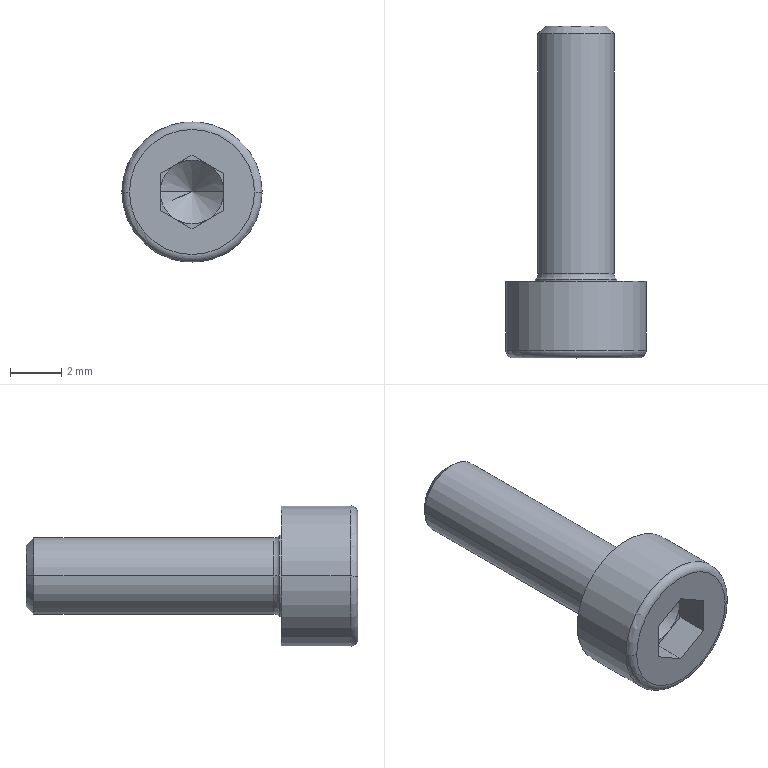Component | SolidWorks | TC_L_12x30_S_0-1_TCL_TCM_12_Screw-1 | 1 solid | 29 faces | box 5.5 x 13 x 5.5 mm | volume 133 mm3 | plane 15 | cylinder 6 | torus 4 | cone 4 | commonest cylinder face diameters 3 x2 3.2 x2 5.5 x2
build123d program:
from build123d import *

# Parameters (mm, degrees)
CUT_EXTRUDE1_DEPTH          = 1.3
SKETCH1_R                   = 2
SKETCH1_R_2                 = 1.6
UNDERHEAD_FILLET_TRIM_DEPTH = 0.4


with BuildPart() as part:
    # Sketch1_2 → Revolve1 (revolve)
    with BuildSketch(Plane.XY, mode=Mode.PRIVATE) as revolve1_sk:
        with BuildLine():
            Line((-3, 0), (-3, 2.45))
            ThreePointArc((-3, 2.45), (-2.912, 2.662), (-2.7, 2.75))
            Line((-2.7, 2.75), (0, 2.75))
            Line((0, 2.75), (0, 1.8))
            ThreePointArc((0, 1.8), (0.08787, 1.588), (0.3, 1.5))
            Line((0.3, 1.5), (9.694, 1.5))
            Line((9.694, 1.5), (10, 1.194))
            Line((10, 1.194), (10, 0))
            Line((10, 0), (-3, 0))
        make_face()
    revolve(revolve1_sk.sketch.rotate(Axis((10, 0, 0), (-1, 0, 0)), 270), axis=Axis((10, 0, 0), (-1, 0, 0)))

    # Sketch2 → Cut-Revolve1 (revolve, cut)
    with BuildSketch(Plane.XY, mode=Mode.PRIVATE) as cut_revolve1_sk:
        Polygon((-3, 0), (-3, 1.25), (-1.7, 1.25), (-0.6, 0), align=None)
    revolve(cut_revolve1_sk.sketch.rotate(Axis((-0.6, 0, 0), (-1, 0, 0)), 270), axis=Axis((-0.6, 0, 0), (-1, 0, 0)), mode=Mode.SUBTRACT)

    # Sketch3 → Cut-Extrude1 (cut)
    with BuildSketch(Plane(origin=(-3, 0, 0), x_dir=(0, 0, -1), z_dir=(1, 0, 0))):
        Polygon((-1.25, 0.7217), (-1.25, -0.7217), (0, -1.443), (1.25, -0.7217), (1.25, 0.7217), (0, 1.443), align=None)
    extrude(amount=CUT_EXTRUDE1_DEPTH, mode=Mode.SUBTRACT)

    # Sketch1 → UnderHead_Fillet_Trim (cut)
    with BuildSketch(Plane(origin=(0, 0, 0), x_dir=(0, 0, -1), z_dir=(1, 0, 0))):
        Circle(SKETCH1_R)
        Circle(SKETCH1_R_2, mode=Mode.SUBTRACT)
    extrude(amount=UNDERHEAD_FILLET_TRIM_DEPTH, mode=Mode.SUBTRACT)


solid = part.part

# Placed as in the assembly
solid = solid.moved(Location((-42, 164.3, 57), (90, 90, 0)))
STEP:
#1=COLOUR_RGB('',0.7922,0.8196,0.9333);
#2=FILL_AREA_STYLE_COLOUR('',#1);
#3=FILL_AREA_STYLE('',(#2));
#4=SURFACE_STYLE_FILL_AREA(#3);
#5=SURFACE_SIDE_STYLE('',(#4));
#6=SURFACE_STYLE_USAGE(.BOTH.,#5);
#7=PRESENTATION_STYLE_ASSIGNMENT((#6));
#8=CARTESIAN_POINT('',(-1.591,6.472,2.244));
#9=VERTEX_POINT('',#8);
#10=CARTESIAN_POINT('',(-1.717,6.472,2.244));
#11=VERTEX_POINT('',#10);
#12=CARTESIAN_POINT('',(-1.654,6.472,2.244));
#13=DIRECTION('',(-0.,1.,0.));
#14=DIRECTION('',(-1.,-0.,0.));
#15=AXIS2_PLACEMENT_3D('',#12,#13,#14);
#16=CIRCLE('',#15,0.06299);
#17=EDGE_CURVE('',#9,#11,#16,.T.);
#18=ORIENTED_EDGE('',*,*,#17,.T.);
#19=CARTESIAN_POINT('',(-1.713,6.48,2.244));
#20=VERTEX_POINT('',#19);
#21=CARTESIAN_POINT('',(-1.724,6.48,2.244));
#22=DIRECTION('',(0.,-0.,1.));
#23=DIRECTION('',(0.,-1.,-0.));
#24=AXIS2_PLACEMENT_3D('',#21,#22,#23);
#25=CIRCLE('',#24,0.01181);
#26=EDGE_CURVE('',#11,#20,#25,.T.);
#27=ORIENTED_EDGE('',*,*,#26,.T.);
#28=CARTESIAN_POINT('',(-1.594,6.48,2.244));
#29=VERTEX_POINT('',#28);
#30=CARTESIAN_POINT('',(-1.654,6.48,2.244));
#31=DIRECTION('',(0.,-1.,-0.));
#32=DIRECTION('',(1.,0.,0.));
#33=AXIS2_PLACEMENT_3D('',#30,#31,#32);
#34=CIRCLE('',#33,0.05906);
#35=EDGE_CURVE('',#20,#29,#34,.T.);
#36=ORIENTED_EDGE('',*,*,#35,.T.);
#37=CARTESIAN_POINT('',(-1.583,6.48,2.244));
#38=DIRECTION('',(-0.,0.,-1.));
#39=DIRECTION('',(0.,1.,0.));
#40=AXIS2_PLACEMENT_3D('',#37,#38,#39);
#41=CIRCLE('',#40,0.01181);
#42=EDGE_CURVE('',#9,#29,#41,.T.);
#43=ORIENTED_EDGE('',*,*,#42,.F.);
#44=EDGE_LOOP('',(#18,#27,#36,#43));
#45=FACE_OUTER_BOUND('',#44,.T.);
#46=CARTESIAN_POINT('',(-1.654,6.48,2.244));
#47=DIRECTION('',(0.,-1.,-0.));
#48=DIRECTION('',(1.,0.,0.));
#49=AXIS2_PLACEMENT_3D('',#46,#47,#48);
#50=TOROIDAL_SURFACE('',#49,0.07087,0.01181);
#51=ADVANCED_FACE('',(#45),#50,.F.);
#52=CARTESIAN_POINT('',(-1.594,6.85,2.244));
#53=VERTEX_POINT('',#52);
#54=CARTESIAN_POINT('',(-1.713,6.85,2.244));
#55=VERTEX_POINT('',#54);
#56=CARTESIAN_POINT('',(-1.654,6.85,2.244));
#57=DIRECTION('',(0.,-1.,-0.));
#58=DIRECTION('',(1.,0.,0.));
#59=AXIS2_PLACEMENT_3D('',#56,#57,#58);
#60=CIRCLE('',#59,0.05906);
#61=EDGE_CURVE('',#53,#55,#60,.T.);
#62=ORIENTED_EDGE('',*,*,#61,.T.);
#63=CARTESIAN_POINT('',(-1.713,6.862,2.244));
#64=DIRECTION('',(0.,-1.,-0.));
#65=VECTOR('',#64,39.37);
#66=LINE('',#63,#65);
#67=EDGE_CURVE('',#55,#20,#66,.T.);
#68=ORIENTED_EDGE('',*,*,#67,.T.);
#69=CARTESIAN_POINT('',(-1.654,6.48,2.244));
#70=DIRECTION('',(0.,-1.,-0.));
#71=DIRECTION('',(1.,0.,0.));
#72=AXIS2_PLACEMENT_3D('',#69,#70,#71);
#73=CIRCLE('',#72,0.05906);
#74=EDGE_CURVE('',#29,#20,#73,.T.);
#75=ORIENTED_EDGE('',*,*,#74,.F.);
#76=CARTESIAN_POINT('',(-1.594,6.862,2.244));
#77=DIRECTION('',(0.,-1.,-0.));
#78=VECTOR('',#77,39.37);
#79=LINE('',#76,#78);
#80=EDGE_CURVE('',#53,#29,#79,.T.);
#81=ORIENTED_EDGE('',*,*,#80,.F.);
#82=EDGE_LOOP('',(#62,#68,#75,#81));
#83=FACE_OUTER_BOUND('',#82,.T.);
#84=CARTESIAN_POINT('',(-1.654,6.862,2.244));
#85=DIRECTION('',(0.,-1.,-0.));
#86=DIRECTION('',(1.,0.,0.));
#87=AXIS2_PLACEMENT_3D('',#84,#85,#86);
#88=CYLINDRICAL_SURFACE('',#87,0.05906);
#89=ADVANCED_FACE('',(#83),#88,.T.);
#90=CARTESIAN_POINT('',(-1.607,6.862,2.244));
#91=VERTEX_POINT('',#90);
#92=CARTESIAN_POINT('',(-1.701,6.862,2.244));
#93=VERTEX_POINT('',#92);
#94=CARTESIAN_POINT('',(-1.654,6.862,2.244));
#95=DIRECTION('',(0.,-1.,-0.));
#96=DIRECTION('',(1.,0.,0.));
#97=AXIS2_PLACEMENT_3D('',#94,#95,#96);
#98=CIRCLE('',#97,0.04699);
#99=EDGE_CURVE('',#91,#93,#98,.T.);
#100=ORIENTED_EDGE('',*,*,#99,.T.);
#101=CARTESIAN_POINT('',(-1.701,6.862,2.244));
#102=DIRECTION('',(-0.7071,-0.7071,-0.));
#103=VECTOR('',#102,39.37);
#104=LINE('',#101,#103);
#105=EDGE_CURVE('',#93,#55,#104,.T.);
#106=ORIENTED_EDGE('',*,*,#105,.T.);
#107=ORIENTED_EDGE('',*,*,#61,.F.);
#108=CARTESIAN_POINT('',(-1.607,6.862,2.244));
#109=DIRECTION('',(0.7071,-0.7071,-0.));
#110=VECTOR('',#109,39.37);
#111=LINE('',#108,#110);
#112=EDGE_CURVE('',#91,#53,#111,.T.);
#113=ORIENTED_EDGE('',*,*,#112,.F.);
#114=EDGE_LOOP('',(#100,#106,#107,#113));
#115=FACE_OUTER_BOUND('',#114,.T.);
#116=CARTESIAN_POINT('',(-1.654,6.862,2.244));
#117=DIRECTION('',(0.,-1.,-0.));
#118=DIRECTION('',(1.,0.,0.));
#119=AXIS2_PLACEMENT_3D('',#116,#117,#118);
#120=CONICAL_SURFACE('',#119,0.04699,0.7854);
#121=ADVANCED_FACE('',(#115),#120,.T.);
#122=CARTESIAN_POINT('',(-1.654,6.472,2.244));
#123=DIRECTION('',(-0.,1.,0.));
#124=DIRECTION('',(-1.,-0.,0.));
#125=AXIS2_PLACEMENT_3D('',#122,#123,#124);
#126=CIRCLE('',#125,0.06299);
#127=EDGE_CURVE('',#11,#9,#126,.T.);
#128=ORIENTED_EDGE('',*,*,#127,.F.);
#129=CARTESIAN_POINT('',(-1.717,6.469,2.244));
#130=VERTEX_POINT('',#129);
#131=CARTESIAN_POINT('',(-1.717,6.484,2.244));
#132=DIRECTION('',(0.,-1.,-0.));
#133=VECTOR('',#132,39.37);
#134=LINE('',#131,#133);
#135=EDGE_CURVE('',#11,#130,#134,.T.);
#136=ORIENTED_EDGE('',*,*,#135,.T.);
#137=CARTESIAN_POINT('',(-1.591,6.469,2.244));
#138=VERTEX_POINT('',#137);
#139=CARTESIAN_POINT('',(-1.654,6.469,2.244));
#140=DIRECTION('',(-0.,1.,0.));
#141=DIRECTION('',(-1.,-0.,0.));
#142=AXIS2_PLACEMENT_3D('',#139,#140,#141);
#143=CIRCLE('',#142,0.06299);
#144=EDGE_CURVE('',#130,#138,#143,.T.);
#145=ORIENTED_EDGE('',*,*,#144,.T.);
#146=CARTESIAN_POINT('',(-1.591,6.484,2.244));
#147=DIRECTION('',(0.,-1.,-0.));
#148=VECTOR('',#147,39.37);
#149=LINE('',#146,#148);
#150=EDGE_CURVE('',#9,#138,#149,.T.);
#151=ORIENTED_EDGE('',*,*,#150,.F.);
#152=EDGE_LOOP('',(#128,#136,#145,#151));
#153=FACE_OUTER_BOUND('',#152,.T.);
#154=CARTESIAN_POINT('',(-1.654,6.484,2.244));
#155=DIRECTION('',(0.,-1.,-0.));
#156=DIRECTION('',(1.,0.,0.));
#157=AXIS2_PLACEMENT_3D('',#154,#155,#156);
#158=CYLINDRICAL_SURFACE('',#157,0.06299);
#159=ADVANCED_FACE('',(#153),#158,.T.);
#160=CARTESIAN_POINT('',(-1.654,6.445,2.244));
#161=VERTEX_POINT('',#160);
#162=CARTESIAN_POINT('',(-1.604,6.402,2.244));
#163=VERTEX_POINT('',#162);
#164=CARTESIAN_POINT('',(-1.654,6.445,2.244));
#165=DIRECTION('',(0.7507,-0.6606,-0.));
#166=VECTOR('',#165,39.37);
#167=LINE('',#164,#166);
#168=EDGE_CURVE('',#161,#163,#167,.T.);
#169=ORIENTED_EDGE('',*,*,#168,.F.);
#170=CARTESIAN_POINT('',(-1.703,6.402,2.244));
#171=VERTEX_POINT('',#170);
#172=CARTESIAN_POINT('',(-1.654,6.445,2.244));
#173=DIRECTION('',(-0.7507,-0.6606,-0.));
#174=VECTOR('',#173,39.37);
#175=LINE('',#172,#174);
#176=EDGE_CURVE('',#161,#171,#175,.T.);
#177=ORIENTED_EDGE('',*,*,#176,.T.);
#178=CARTESIAN_POINT('',(-1.678,6.402,2.201));
#179=VERTEX_POINT('',#178);
#180=CARTESIAN_POINT('',(-1.654,6.402,2.244));
#181=DIRECTION('',(0.,-1.,-0.));
#182=DIRECTION('',(1.,0.,0.));
#183=AXIS2_PLACEMENT_3D('',#180,#181,#182);
#184=CIRCLE('',#183,0.04921);
#185=EDGE_CURVE('',#171,#179,#184,.T.);
#186=ORIENTED_EDGE('',*,*,#185,.T.);
#187=CARTESIAN_POINT('',(-1.629,6.402,2.201));
#188=VERTEX_POINT('',#187);
#189=CARTESIAN_POINT('',(-1.654,6.402,2.244));
#190=DIRECTION('',(0.,-1.,-0.));
#191=DIRECTION('',(1.,0.,0.));
#192=AXIS2_PLACEMENT_3D('',#189,#190,#191);
#193=CIRCLE('',#192,0.04921);
#194=EDGE_CURVE('',#179,#188,#193,.T.);
#195=ORIENTED_EDGE('',*,*,#194,.T.);
#196=CARTESIAN_POINT('',(-1.654,6.402,2.244));
#197=DIRECTION('',(0.,-1.,-0.));
#198=DIRECTION('',(1.,0.,0.));
#199=AXIS2_PLACEMENT_3D('',#196,#197,#198);
#200=CIRCLE('',#199,0.04921);
#201=EDGE_CURVE('',#188,#163,#200,.T.);
#202=ORIENTED_EDGE('',*,*,#201,.T.);
#203=EDGE_LOOP('',(#169,#177,#186,#195,#202));
#204=FACE_OUTER_BOUND('',#203,.T.);
#205=CARTESIAN_POINT('',(-1.654,-32.925,2.244));
#206=DIRECTION('',(0.,-1.,-0.));
#207=DIRECTION('',(1.,0.,-0.));
#208=AXIS2_PLACEMENT_3D('',#205,#206,#207);
#209=CONICAL_SURFACE('',#208,44.739,0.8491);
#210=ADVANCED_FACE('',(#204),#209,.F.);
#211=CARTESIAN_POINT('',(-1.545,6.469,2.244));
#212=VERTEX_POINT('',#211);
#213=CARTESIAN_POINT('',(-1.762,6.469,2.244));
#214=VERTEX_POINT('',#213);
#215=CARTESIAN_POINT('',(-1.654,6.469,2.244));
#216=DIRECTION('',(0.,-1.,-0.));
#217=DIRECTION('',(1.,0.,0.));
#218=AXIS2_PLACEMENT_3D('',#215,#216,#217);
#219=CIRCLE('',#218,0.1083);
#220=EDGE_CURVE('',#212,#214,#219,.T.);
#221=ORIENTED_EDGE('',*,*,#220,.T.);
#222=CARTESIAN_POINT('',(-1.762,6.362,2.244));
#223=VERTEX_POINT('',#222);
#224=CARTESIAN_POINT('',(-1.762,6.862,2.244));
#225=DIRECTION('',(0.,-1.,-0.));
#226=VECTOR('',#225,39.37);
#227=LINE('',#224,#226);
#228=EDGE_CURVE('',#214,#223,#227,.T.);
#229=ORIENTED_EDGE('',*,*,#228,.T.);
#230=CARTESIAN_POINT('',(-1.545,6.362,2.244));
#231=VERTEX_POINT('',#230);
#232=CARTESIAN_POINT('',(-1.654,6.362,2.244));
#233=DIRECTION('',(0.,-1.,-0.));
#234=DIRECTION('',(1.,0.,0.));
#235=AXIS2_PLACEMENT_3D('',#232,#233,#234);
#236=CIRCLE('',#235,0.1083);
#237=EDGE_CURVE('',#231,#223,#236,.T.);
#238=ORIENTED_EDGE('',*,*,#237,.F.);
#239=CARTESIAN_POINT('',(-1.545,6.862,2.244));
#240=DIRECTION('',(0.,-1.,-0.));
#241=VECTOR('',#240,39.37);
#242=LINE('',#239,#241);
#243=EDGE_CURVE('',#212,#231,#242,.T.);
#244=ORIENTED_EDGE('',*,*,#243,.F.);
#245=EDGE_LOOP('',(#221,#229,#238,#244));
#246=FACE_OUTER_BOUND('',#245,.T.);
#247=CARTESIAN_POINT('',(-1.654,6.862,2.244));
#248=DIRECTION('',(0.,-1.,-0.));
#249=DIRECTION('',(1.,0.,0.));
#250=AXIS2_PLACEMENT_3D('',#247,#248,#249);
#251=CYLINDRICAL_SURFACE('',#250,0.1083);
#252=ADVANCED_FACE('',(#246),#251,.T.);
#253=ORIENTED_EDGE('',*,*,#237,.T.);
#254=CARTESIAN_POINT('',(-1.75,6.35,2.244));
#255=VERTEX_POINT('',#254);
#256=CARTESIAN_POINT('',(-1.75,6.362,2.244));
#257=DIRECTION('',(0.,-0.,1.));
#258=DIRECTION('',(0.,-1.,-0.));
#259=AXIS2_PLACEMENT_3D('',#256,#257,#258);
#260=CIRCLE('',#259,0.01181);
#261=EDGE_CURVE('',#223,#255,#260,.T.);
#262=ORIENTED_EDGE('',*,*,#261,.T.);
#263=CARTESIAN_POINT('',(-1.557,6.35,2.244));
#264=VERTEX_POINT('',#263);
#265=CARTESIAN_POINT('',(-1.654,6.35,2.244));
#266=DIRECTION('',(0.,-1.,-0.));
#267=DIRECTION('',(1.,0.,0.));
#268=AXIS2_PLACEMENT_3D('',#265,#266,#267);
#269=CIRCLE('',#268,0.09646);
#270=EDGE_CURVE('',#264,#255,#269,.T.);
#271=ORIENTED_EDGE('',*,*,#270,.F.);
#272=CARTESIAN_POINT('',(-1.557,6.362,2.244));
#273=DIRECTION('',(-0.,0.,-1.));
#274=DIRECTION('',(0.,1.,0.));
#275=AXIS2_PLACEMENT_3D('',#272,#273,#274);
#276=CIRCLE('',#275,0.01181);
#277=EDGE_CURVE('',#231,#264,#276,.T.);
#278=ORIENTED_EDGE('',*,*,#277,.F.);
#279=EDGE_LOOP('',(#253,#262,#271,#278));
#280=FACE_OUTER_BOUND('',#279,.T.);
#281=CARTESIAN_POINT('',(-1.654,6.362,2.244));
#282=DIRECTION('',(0.,-1.,-0.));
#283=DIRECTION('',(1.,0.,0.));
#284=AXIS2_PLACEMENT_3D('',#281,#282,#283);
#285=TOROIDAL_SURFACE('',#284,0.09646,0.01181);
#286=ADVANCED_FACE('',(#280),#285,.T.);
#287=ORIENTED_EDGE('',*,*,#270,.T.);
#288=CARTESIAN_POINT('',(-1.654,6.35,2.244));
#289=DIRECTION('',(0.,-1.,-0.));
#290=DIRECTION('',(1.,0.,0.));
#291=AXIS2_PLACEMENT_3D('',#288,#289,#290);
#292=CIRCLE('',#291,0.09646);
#293=EDGE_CURVE('',#255,#264,#292,.T.);
#294=ORIENTED_EDGE('',*,*,#293,.T.);
#295=EDGE_LOOP('',(#287,#294));
#296=FACE_OUTER_BOUND('',#295,.T.);
#297=CARTESIAN_POINT('',(-1.604,6.35,2.216));
#298=VERTEX_POINT('',#297);
#299=CARTESIAN_POINT('',(-1.654,6.35,2.187));
#300=VERTEX_POINT('',#299);
#301=CARTESIAN_POINT('',(-1.604,6.35,2.216));
#302=DIRECTION('',(-0.866,-0.,-0.5));
#303=VECTOR('',#302,39.37);
#304=LINE('',#301,#303);
#305=EDGE_CURVE('',#298,#300,#304,.T.);
#306=ORIENTED_EDGE('',*,*,#305,.T.);
#307=CARTESIAN_POINT('',(-1.703,6.35,2.216));
#308=VERTEX_POINT('',#307);
#309=CARTESIAN_POINT('',(-1.654,6.35,2.187));
#310=DIRECTION('',(-0.866,-0.,0.5));
#311=VECTOR('',#310,39.37);
#312=LINE('',#309,#311);
#313=EDGE_CURVE('',#300,#308,#312,.T.);
#314=ORIENTED_EDGE('',*,*,#313,.T.);
#315=CARTESIAN_POINT('',(-1.703,6.35,2.273));
#316=VERTEX_POINT('',#315);
#317=CARTESIAN_POINT('',(-1.703,6.35,2.216));
#318=DIRECTION('',(0.,-0.,1.));
#319=VECTOR('',#318,39.37);
#320=LINE('',#317,#319);
#321=EDGE_CURVE('',#308,#316,#320,.T.);
#322=ORIENTED_EDGE('',*,*,#321,.T.);
#323=CARTESIAN_POINT('',(-1.654,6.35,2.301));
#324=VERTEX_POINT('',#323);
#325=CARTESIAN_POINT('',(-1.703,6.35,2.273));
#326=DIRECTION('',(0.866,0.,0.5));
#327=VECTOR('',#326,39.37);
#328=LINE('',#325,#327);
#329=EDGE_CURVE('',#316,#324,#328,.T.);
#330=ORIENTED_EDGE('',*,*,#329,.T.);
#331=CARTESIAN_POINT('',(-1.604,6.35,2.273));
#332=VERTEX_POINT('',#331);
#333=CARTESIAN_POINT('',(-1.654,6.35,2.301));
#334=DIRECTION('',(0.866,0.,-0.5));
#335=VECTOR('',#334,39.37);
#336=LINE('',#333,#335);
#337=EDGE_CURVE('',#324,#332,#336,.T.);
#338=ORIENTED_EDGE('',*,*,#337,.T.);
#339=CARTESIAN_POINT('',(-1.604,6.35,2.273));
#340=DIRECTION('',(-0.,0.,-1.));
#341=VECTOR('',#340,39.37);
#342=LINE('',#339,#341);
#343=EDGE_CURVE('',#332,#298,#342,.T.);
#344=ORIENTED_EDGE('',*,*,#343,.T.);
#345=EDGE_LOOP('',(#306,#314,#322,#330,#338,#344));
#346=FACE_BOUND('',#345,.T.);
#347=CARTESIAN_POINT('',(-1.654,6.35,2.244));
#348=DIRECTION('',(-0.,1.,0.));
#349=DIRECTION('',(-1.,-0.,0.));
#350=AXIS2_PLACEMENT_3D('',#347,#348,#349);
#351=PLANE('',#350);
#352=ADVANCED_FACE('',(#296,#346),#351,.F.);
#353=ORIENTED_EDGE('',*,*,#261,.F.);
#354=CARTESIAN_POINT('',(-1.654,6.362,2.244));
#355=DIRECTION('',(0.,-1.,-0.));
#356=DIRECTION('',(1.,0.,0.));
#357=AXIS2_PLACEMENT_3D('',#354,#355,#356);
#358=CIRCLE('',#357,0.1083);
#359=EDGE_CURVE('',#223,#231,#358,.T.);
#360=ORIENTED_EDGE('',*,*,#359,.T.);
#361=ORIENTED_EDGE('',*,*,#277,.T.);
#362=ORIENTED_EDGE('',*,*,#293,.F.);
#363=EDGE_LOOP('',(#353,#360,#361,#362));
#364=FACE_OUTER_BOUND('',#363,.T.);
#365=CARTESIAN_POINT('',(-1.654,6.362,2.244));
#366=DIRECTION('',(0.,-1.,-0.));
#367=DIRECTION('',(1.,0.,0.));
#368=AXIS2_PLACEMENT_3D('',#365,#366,#367);
#369=TOROIDAL_SURFACE('',#368,0.09646,0.01181);
#370=ADVANCED_FACE('',(#364),#369,.T.);
#371=ORIENTED_EDGE('',*,*,#228,.F.);
#372=CARTESIAN_POINT('',(-1.654,6.469,2.244));
#373=DIRECTION('',(0.,-1.,-0.));
#374=DIRECTION('',(1.,0.,0.));
#375=AXIS2_PLACEMENT_3D('',#372,#373,#374);
#376=CIRCLE('',#375,0.1083);
#377=EDGE_CURVE('',#214,#212,#376,.T.);
#378=ORIENTED_EDGE('',*,*,#377,.T.);
#379=ORIENTED_EDGE('',*,*,#243,.T.);
#380=ORIENTED_EDGE('',*,*,#359,.F.);
#381=EDGE_LOOP('',(#371,#378,#379,#380));
#382=FACE_OUTER_BOUND('',#381,.T.);
#383=CARTESIAN_POINT('',(-1.654,6.862,2.244));
#384=DIRECTION('',(0.,-1.,-0.));
#385=DIRECTION('',(1.,0.,0.));
#386=AXIS2_PLACEMENT_3D('',#383,#384,#385);
#387=CYLINDRICAL_SURFACE('',#386,0.1083);
#388=ADVANCED_FACE('',(#382),#387,.T.);
#389=ORIENTED_EDGE('',*,*,#220,.F.);
#390=ORIENTED_EDGE('',*,*,#377,.F.);
#391=EDGE_LOOP('',(#389,#390));
#392=FACE_OUTER_BOUND('',#391,.T.);
#393=CARTESIAN_POINT('',(-1.654,6.469,2.244));
#394=DIRECTION('',(-0.,1.,0.));
#395=DIRECTION('',(-1.,-0.,0.));
#396=AXIS2_PLACEMENT_3D('',#393,#394,#395);
#397=CIRCLE('',#396,0.06299);
#398=EDGE_CURVE('',#138,#130,#397,.T.);
#399=ORIENTED_EDGE('',*,*,#398,.F.);
#400=ORIENTED_EDGE('',*,*,#144,.F.);
#401=EDGE_LOOP('',(#399,#400));
#402=FACE_BOUND('',#401,.T.);
#403=CARTESIAN_POINT('',(-1.654,6.469,2.352));
#404=DIRECTION('',(0.,-1.,-0.));
#405=DIRECTION('',(1.,0.,-0.));
#406=AXIS2_PLACEMENT_3D('',#403,#404,#405);
#407=PLANE('',#406);
#408=ADVANCED_FACE('',(#392,#402),#407,.F.);
#409=CARTESIAN_POINT('',(-1.654,6.402,2.301));
#410=VERTEX_POINT('',#409);
#411=CARTESIAN_POINT('',(-1.629,6.402,2.287));
#412=VERTEX_POINT('',#411);
#413=CARTESIAN_POINT('',(-1.654,6.402,2.301));
#414=DIRECTION('',(0.866,0.,-0.5));
#415=VECTOR('',#414,39.37);
#416=LINE('',#413,#415);
#417=EDGE_CURVE('',#410,#412,#416,.T.);
#418=ORIENTED_EDGE('',*,*,#417,.T.);
#419=CARTESIAN_POINT('',(-1.604,6.402,2.273));
#420=VERTEX_POINT('',#419);
#421=CARTESIAN_POINT('',(-1.654,6.402,2.301));
#422=DIRECTION('',(0.866,0.,-0.5));
#423=VECTOR('',#422,39.37);
#424=LINE('',#421,#423);
#425=EDGE_CURVE('',#412,#420,#424,.T.);
#426=ORIENTED_EDGE('',*,*,#425,.T.);
#427=CARTESIAN_POINT('',(-1.604,6.402,2.273));
#428=DIRECTION('',(0.,-1.,-0.));
#429=VECTOR('',#428,39.37);
#430=LINE('',#427,#429);
#431=EDGE_CURVE('',#420,#332,#430,.T.);
#432=ORIENTED_EDGE('',*,*,#431,.T.);
#433=ORIENTED_EDGE('',*,*,#337,.F.);
#434=CARTESIAN_POINT('',(-1.654,6.402,2.301));
#435=DIRECTION('',(0.,-1.,-0.));
#436=VECTOR('',#435,39.37);
#437=LINE('',#434,#436);
#438=EDGE_CURVE('',#410,#324,#437,.T.);
#439=ORIENTED_EDGE('',*,*,#438,.F.);
#440=EDGE_LOOP('',(#418,#426,#432,#433,#439));
#441=FACE_OUTER_BOUND('',#440,.T.);
#442=CARTESIAN_POINT('',(-1.654,6.402,2.301));
#443=DIRECTION('',(-0.5,0.,-0.866));
#444=DIRECTION('',(-0.866,-0.,0.5));
#445=AXIS2_PLACEMENT_3D('',#442,#443,#444);
#446=PLANE('',#445);
#447=ADVANCED_FACE('',(#441),#446,.T.);
#448=CARTESIAN_POINT('',(-1.604,6.402,2.273));
#449=DIRECTION('',(-0.,0.,-1.));
#450=VECTOR('',#449,39.37);
#451=LINE('',#448,#450);
#452=EDGE_CURVE('',#420,#163,#451,.T.);
#453=ORIENTED_EDGE('',*,*,#452,.T.);
#454=CARTESIAN_POINT('',(-1.604,6.402,2.216));
#455=VERTEX_POINT('',#454);
#456=CARTESIAN_POINT('',(-1.604,6.402,2.273));
#457=DIRECTION('',(-0.,0.,-1.));
#458=VECTOR('',#457,39.37);
#459=LINE('',#456,#458);
#460=EDGE_CURVE('',#163,#455,#459,.T.);
#461=ORIENTED_EDGE('',*,*,#460,.T.);
#462=CARTESIAN_POINT('',(-1.604,6.402,2.216));
#463=DIRECTION('',(0.,-1.,-0.));
#464=VECTOR('',#463,39.37);
#465=LINE('',#462,#464);
#466=EDGE_CURVE('',#455,#298,#465,.T.);
#467=ORIENTED_EDGE('',*,*,#466,.T.);
#468=ORIENTED_EDGE('',*,*,#343,.F.);
#469=ORIENTED_EDGE('',*,*,#431,.F.);
#470=EDGE_LOOP('',(#453,#461,#467,#468,#469));
#471=FACE_OUTER_BOUND('',#470,.T.);
#472=CARTESIAN_POINT('',(-1.604,6.402,2.273));
#473=DIRECTION('',(-1.,-0.,0.));
#474=DIRECTION('',(0.,-1.,-0.));
#475=AXIS2_PLACEMENT_3D('',#472,#473,#474);
#476=PLANE('',#475);
#477=ADVANCED_FACE('',(#471),#476,.T.);
#478=CARTESIAN_POINT('',(-1.604,6.402,2.216));
#479=DIRECTION('',(-0.866,-0.,-0.5));
#480=VECTOR('',#479,39.37);
#481=LINE('',#478,#480);
#482=EDGE_CURVE('',#455,#188,#481,.T.);
#483=ORIENTED_EDGE('',*,*,#482,.T.);
#484=CARTESIAN_POINT('',(-1.654,6.402,2.187));
#485=VERTEX_POINT('',#484);
#486=CARTESIAN_POINT('',(-1.604,6.402,2.216));
#487=DIRECTION('',(-0.866,-0.,-0.5));
#488=VECTOR('',#487,39.37);
#489=LINE('',#486,#488);
#490=EDGE_CURVE('',#188,#485,#489,.T.);
#491=ORIENTED_EDGE('',*,*,#490,.T.);
#492=CARTESIAN_POINT('',(-1.654,6.402,2.187));
#493=DIRECTION('',(0.,-1.,-0.));
#494=VECTOR('',#493,39.37);
#495=LINE('',#492,#494);
#496=EDGE_CURVE('',#485,#300,#495,.T.);
#497=ORIENTED_EDGE('',*,*,#496,.T.);
#498=ORIENTED_EDGE('',*,*,#305,.F.);
#499=ORIENTED_EDGE('',*,*,#466,.F.);
#500=EDGE_LOOP('',(#483,#491,#497,#498,#499));
#501=FACE_OUTER_BOUND('',#500,.T.);
#502=CARTESIAN_POINT('',(-1.604,6.402,2.216));
#503=DIRECTION('',(-0.5,-0.,0.866));
#504=DIRECTION('',(0.866,0.,0.5));
#505=AXIS2_PLACEMENT_3D('',#502,#503,#504);
#506=PLANE('',#505);
#507=ADVANCED_FACE('',(#501),#506,.T.);
#508=CARTESIAN_POINT('',(-1.654,6.402,2.187));
#509=DIRECTION('',(-0.866,-0.,0.5));
#510=VECTOR('',#509,39.37);
#511=LINE('',#508,#510);
#512=EDGE_CURVE('',#485,#179,#511,.T.);
#513=ORIENTED_EDGE('',*,*,#512,.T.);
#514=CARTESIAN_POINT('',(-1.703,6.402,2.216));
#515=VERTEX_POINT('',#514);
#516=CARTESIAN_POINT('',(-1.654,6.402,2.187));
#517=DIRECTION('',(-0.866,-0.,0.5));
#518=VECTOR('',#517,39.37);
#519=LINE('',#516,#518);
#520=EDGE_CURVE('',#179,#515,#519,.T.);
#521=ORIENTED_EDGE('',*,*,#520,.T.);
#522=CARTESIAN_POINT('',(-1.703,6.402,2.216));
#523=DIRECTION('',(0.,-1.,-0.));
#524=VECTOR('',#523,39.37);
#525=LINE('',#522,#524);
#526=EDGE_CURVE('',#515,#308,#525,.T.);
#527=ORIENTED_EDGE('',*,*,#526,.T.);
#528=ORIENTED_EDGE('',*,*,#313,.F.);
#529=ORIENTED_EDGE('',*,*,#496,.F.);
#530=EDGE_LOOP('',(#513,#521,#527,#528,#529));
#531=FACE_OUTER_BOUND('',#530,.T.);
#532=CARTESIAN_POINT('',(-1.654,6.402,2.187));
#533=DIRECTION('',(0.5,-0.,0.866));
#534=DIRECTION('',(0.866,0.,-0.5));
#535=AXIS2_PLACEMENT_3D('',#532,#533,#534);
#536=PLANE('',#535);
#537=ADVANCED_FACE('',(#531),#536,.T.);
#538=CARTESIAN_POINT('',(-1.703,6.402,2.216));
#539=DIRECTION('',(0.,-0.,1.));
#540=VECTOR('',#539,39.37);
#541=LINE('',#538,#540);
#542=EDGE_CURVE('',#515,#171,#541,.T.);
#543=ORIENTED_EDGE('',*,*,#542,.T.);
#544=CARTESIAN_POINT('',(-1.703,6.402,2.273));
#545=VERTEX_POINT('',#544);
#546=CARTESIAN_POINT('',(-1.703,6.402,2.216));
#547=DIRECTION('',(0.,-0.,1.));
#548=VECTOR('',#547,39.37);
#549=LINE('',#546,#548);
#550=EDGE_CURVE('',#171,#545,#549,.T.);
#551=ORIENTED_EDGE('',*,*,#550,.T.);
#552=CARTESIAN_POINT('',(-1.703,6.402,2.273));
#553=DIRECTION('',(0.,-1.,-0.));
#554=VECTOR('',#553,39.37);
#555=LINE('',#552,#554);
#556=EDGE_CURVE('',#545,#316,#555,.T.);
#557=ORIENTED_EDGE('',*,*,#556,.T.);
#558=ORIENTED_EDGE('',*,*,#321,.F.);
#559=ORIENTED_EDGE('',*,*,#526,.F.);
#560=EDGE_LOOP('',(#543,#551,#557,#558,#559));
#561=FACE_OUTER_BOUND('',#560,.T.);
#562=CARTESIAN_POINT('',(-1.703,6.402,2.216));
#563=DIRECTION('',(1.,0.,-0.));
#564=DIRECTION('',(-0.,1.,0.));
#565=AXIS2_PLACEMENT_3D('',#562,#563,#564);
#566=PLANE('',#565);
#567=ADVANCED_FACE('',(#561),#566,.T.);
#568=CARTESIAN_POINT('',(-1.678,6.402,2.287));
#569=VERTEX_POINT('',#568);
#570=CARTESIAN_POINT('',(-1.703,6.402,2.273));
#571=DIRECTION('',(0.866,0.,0.5));
#572=VECTOR('',#571,39.37);
#573=LINE('',#570,#572);
#574=EDGE_CURVE('',#545,#569,#573,.T.);
#575=ORIENTED_EDGE('',*,*,#574,.T.);
#576=CARTESIAN_POINT('',(-1.703,6.402,2.273));
#577=DIRECTION('',(0.866,0.,0.5));
#578=VECTOR('',#577,39.37);
#579=LINE('',#576,#578);
#580=EDGE_CURVE('',#569,#410,#579,.T.);
#581=ORIENTED_EDGE('',*,*,#580,.T.);
#582=ORIENTED_EDGE('',*,*,#438,.T.);
#583=ORIENTED_EDGE('',*,*,#329,.F.);
#584=ORIENTED_EDGE('',*,*,#556,.F.);
#585=EDGE_LOOP('',(#575,#581,#582,#583,#584));
#586=FACE_OUTER_BOUND('',#585,.T.);
#587=CARTESIAN_POINT('',(-1.703,6.402,2.273));
#588=DIRECTION('',(0.5,0.,-0.866));
#589=DIRECTION('',(-0.866,-0.,-0.5));
#590=AXIS2_PLACEMENT_3D('',#587,#588,#589);
#591=PLANE('',#590);
#592=ADVANCED_FACE('',(#586),#591,.T.);
#593=CARTESIAN_POINT('',(-1.654,6.402,2.244));
#594=DIRECTION('',(0.,-1.,-0.));
#595=DIRECTION('',(1.,0.,0.));
#596=AXIS2_PLACEMENT_3D('',#593,#594,#595);
#597=CIRCLE('',#596,0.04921);
#598=EDGE_CURVE('',#569,#171,#597,.T.);
#599=ORIENTED_EDGE('',*,*,#598,.F.);
#600=ORIENTED_EDGE('',*,*,#574,.F.);
#601=ORIENTED_EDGE('',*,*,#550,.F.);
#602=EDGE_LOOP('',(#599,#600,#601));
#603=FACE_OUTER_BOUND('',#602,.T.);
#604=CARTESIAN_POINT('',(-1.654,6.402,2.244));
#605=DIRECTION('',(-0.,1.,0.));
#606=DIRECTION('',(-1.,-0.,0.));
#607=AXIS2_PLACEMENT_3D('',#604,#605,#606);
#608=PLANE('',#607);
#609=ADVANCED_FACE('',(#603),#608,.F.);
#610=CARTESIAN_POINT('',(-1.654,6.402,2.244));
#611=DIRECTION('',(0.,-1.,-0.));
#612=DIRECTION('',(1.,0.,0.));
#613=AXIS2_PLACEMENT_3D('',#610,#611,#612);
#614=CIRCLE('',#613,0.04921);
#615=EDGE_CURVE('',#412,#569,#614,.T.);
#616=ORIENTED_EDGE('',*,*,#615,.F.);
#617=ORIENTED_EDGE('',*,*,#417,.F.);
#618=ORIENTED_EDGE('',*,*,#580,.F.);
#619=EDGE_LOOP('',(#616,#617,#618));
#620=FACE_OUTER_BOUND('',#619,.T.);
#621=CARTESIAN_POINT('',(-1.654,6.402,2.244));
#622=DIRECTION('',(-0.,1.,0.));
#623=DIRECTION('',(-1.,-0.,0.));
#624=AXIS2_PLACEMENT_3D('',#621,#622,#623);
#625=PLANE('',#624);
#626=ADVANCED_FACE('',(#620),#625,.F.);
#627=CARTESIAN_POINT('',(-1.654,6.402,2.244));
#628=DIRECTION('',(0.,-1.,-0.));
#629=DIRECTION('',(1.,0.,0.));
#630=AXIS2_PLACEMENT_3D('',#627,#628,#629);
#631=CIRCLE('',#630,0.04921);
#632=EDGE_CURVE('',#163,#412,#631,.T.);
#633=ORIENTED_EDGE('',*,*,#632,.F.);
#634=ORIENTED_EDGE('',*,*,#452,.F.);
#635=ORIENTED_EDGE('',*,*,#425,.F.);
#636=EDGE_LOOP('',(#633,#634,#635));
#637=FACE_OUTER_BOUND('',#636,.T.);
#638=CARTESIAN_POINT('',(-1.654,6.402,2.244));
#639=DIRECTION('',(-0.,1.,0.));
#640=DIRECTION('',(-1.,-0.,0.));
#641=AXIS2_PLACEMENT_3D('',#638,#639,#640);
#642=PLANE('',#641);
#643=ADVANCED_FACE('',(#637),#642,.F.);
#644=ORIENTED_EDGE('',*,*,#201,.F.);
#645=ORIENTED_EDGE('',*,*,#482,.F.);
#646=ORIENTED_EDGE('',*,*,#460,.F.);
#647=EDGE_LOOP('',(#644,#645,#646));
#648=FACE_OUTER_BOUND('',#647,.T.);
#649=CARTESIAN_POINT('',(-1.654,6.402,2.244));
#650=DIRECTION('',(-0.,1.,0.));
#651=DIRECTION('',(-1.,-0.,0.));
#652=AXIS2_PLACEMENT_3D('',#649,#650,#651);
#653=PLANE('',#652);
#654=ADVANCED_FACE('',(#648),#653,.F.);
#655=ORIENTED_EDGE('',*,*,#194,.F.);
#656=ORIENTED_EDGE('',*,*,#512,.F.);
#657=ORIENTED_EDGE('',*,*,#490,.F.);
#658=EDGE_LOOP('',(#655,#656,#657));
#659=FACE_OUTER_BOUND('',#658,.T.);
#660=CARTESIAN_POINT('',(-1.654,6.402,2.244));
#661=DIRECTION('',(-0.,1.,0.));
#662=DIRECTION('',(-1.,-0.,0.));
#663=AXIS2_PLACEMENT_3D('',#660,#661,#662);
#664=PLANE('',#663);
#665=ADVANCED_FACE('',(#659),#664,.F.);
#666=ORIENTED_EDGE('',*,*,#185,.F.);
#667=ORIENTED_EDGE('',*,*,#542,.F.);
#668=ORIENTED_EDGE('',*,*,#520,.F.);
#669=EDGE_LOOP('',(#666,#667,#668));
#670=FACE_OUTER_BOUND('',#669,.T.);
#671=CARTESIAN_POINT('',(-1.654,6.402,2.244));
#672=DIRECTION('',(-0.,1.,0.));
#673=DIRECTION('',(-1.,-0.,0.));
#674=AXIS2_PLACEMENT_3D('',#671,#672,#673);
#675=PLANE('',#674);
#676=ADVANCED_FACE('',(#670),#675,.F.);
#677=ORIENTED_EDGE('',*,*,#176,.F.);
#678=ORIENTED_EDGE('',*,*,#168,.T.);
#679=ORIENTED_EDGE('',*,*,#632,.T.);
#680=ORIENTED_EDGE('',*,*,#615,.T.);
#681=ORIENTED_EDGE('',*,*,#598,.T.);
#682=EDGE_LOOP('',(#677,#678,#679,#680,#681));
#683=FACE_OUTER_BOUND('',#682,.T.);
#684=CARTESIAN_POINT('',(-1.654,-32.925,2.244));
#685=DIRECTION('',(0.,-1.,-0.));
#686=DIRECTION('',(1.,0.,-0.));
#687=AXIS2_PLACEMENT_3D('',#684,#685,#686);
#688=CONICAL_SURFACE('',#687,44.739,0.8491);
#689=ADVANCED_FACE('',(#683),#688,.F.);
#690=ORIENTED_EDGE('',*,*,#135,.F.);
#691=ORIENTED_EDGE('',*,*,#17,.F.);
#692=ORIENTED_EDGE('',*,*,#150,.T.);
#693=ORIENTED_EDGE('',*,*,#398,.T.);
#694=EDGE_LOOP('',(#690,#691,#692,#693));
#695=FACE_OUTER_BOUND('',#694,.T.);
#696=CARTESIAN_POINT('',(-1.654,6.484,2.244));
#697=DIRECTION('',(0.,-1.,-0.));
#698=DIRECTION('',(1.,0.,0.));
#699=AXIS2_PLACEMENT_3D('',#696,#697,#698);
#700=CYLINDRICAL_SURFACE('',#699,0.06299);
#701=ADVANCED_FACE('',(#695),#700,.T.);
#702=ORIENTED_EDGE('',*,*,#99,.F.);
#703=CARTESIAN_POINT('',(-1.654,6.862,2.244));
#704=DIRECTION('',(0.,-1.,-0.));
#705=DIRECTION('',(1.,0.,0.));
#706=AXIS2_PLACEMENT_3D('',#703,#704,#705);
#707=CIRCLE('',#706,0.04699);
#708=EDGE_CURVE('',#93,#91,#707,.T.);
#709=ORIENTED_EDGE('',*,*,#708,.F.);
#710=EDGE_LOOP('',(#702,#709));
#711=FACE_OUTER_BOUND('',#710,.T.);
#712=CARTESIAN_POINT('',(-1.654,6.862,2.291));
#713=DIRECTION('',(0.,-1.,-0.));
#714=DIRECTION('',(1.,0.,-0.));
#715=AXIS2_PLACEMENT_3D('',#712,#713,#714);
#716=PLANE('',#715);
#717=ADVANCED_FACE('',(#711),#716,.F.);
#718=ORIENTED_EDGE('',*,*,#105,.F.);
#719=ORIENTED_EDGE('',*,*,#708,.T.);
#720=ORIENTED_EDGE('',*,*,#112,.T.);
#721=CARTESIAN_POINT('',(-1.654,6.85,2.244));
#722=DIRECTION('',(0.,-1.,-0.));
#723=DIRECTION('',(1.,0.,0.));
#724=AXIS2_PLACEMENT_3D('',#721,#722,#723);
#725=CIRCLE('',#724,0.05906);
#726=EDGE_CURVE('',#55,#53,#725,.T.);
#727=ORIENTED_EDGE('',*,*,#726,.F.);
#728=EDGE_LOOP('',(#718,#719,#720,#727));
#729=FACE_OUTER_BOUND('',#728,.T.);
#730=CARTESIAN_POINT('',(-1.654,6.862,2.244));
#731=DIRECTION('',(0.,-1.,-0.));
#732=DIRECTION('',(1.,0.,0.));
#733=AXIS2_PLACEMENT_3D('',#730,#731,#732);
#734=CONICAL_SURFACE('',#733,0.04699,0.7854);
#735=ADVANCED_FACE('',(#729),#734,.T.);
#736=ORIENTED_EDGE('',*,*,#67,.F.);
#737=ORIENTED_EDGE('',*,*,#726,.T.);
#738=ORIENTED_EDGE('',*,*,#80,.T.);
#739=ORIENTED_EDGE('',*,*,#35,.F.);
#740=EDGE_LOOP('',(#736,#737,#738,#739));
#741=FACE_OUTER_BOUND('',#740,.T.);
#742=CARTESIAN_POINT('',(-1.654,6.862,2.244));
#743=DIRECTION('',(0.,-1.,-0.));
#744=DIRECTION('',(1.,0.,0.));
#745=AXIS2_PLACEMENT_3D('',#742,#743,#744);
#746=CYLINDRICAL_SURFACE('',#745,0.05906);
#747=ADVANCED_FACE('',(#741),#746,.T.);
#748=ORIENTED_EDGE('',*,*,#26,.F.);
#749=ORIENTED_EDGE('',*,*,#127,.T.);
#750=ORIENTED_EDGE('',*,*,#42,.T.);
#751=ORIENTED_EDGE('',*,*,#74,.T.);
#752=EDGE_LOOP('',(#748,#749,#750,#751));
#753=FACE_OUTER_BOUND('',#752,.T.);
#754=CARTESIAN_POINT('',(-1.654,6.48,2.244));
#755=DIRECTION('',(0.,-1.,-0.));
#756=DIRECTION('',(1.,0.,0.));
#757=AXIS2_PLACEMENT_3D('',#754,#755,#756);
#758=TOROIDAL_SURFACE('',#757,0.07087,0.01181);
#759=ADVANCED_FACE('',(#753),#758,.F.);
#760=CLOSED_SHELL('',(#51,#89,#121,#159,#210,#252,#286,#352,#370,#388,#408,#447,#477,#507,#537,#567,#592,#609,#626,#643,#654,#665,#676,#689,#701,#717,#735,#747,#759));
#761=MANIFOLD_SOLID_BREP('',#760);
#762=STYLED_ITEM('',(#7),#761);
#763=(LENGTH_UNIT()NAMED_UNIT(*)SI_UNIT($,.METRE.));
#764=LENGTH_MEASURE_WITH_UNIT(LENGTH_MEASURE(0.0254),#763);
#765=DIMENSIONAL_EXPONENTS(1.,0.,0.,0.,0.,0.,0.);
#766=(CONVERSION_BASED_UNIT('',#764)LENGTH_UNIT()NAMED_UNIT(#765));
#767=UNCERTAINTY_MEASURE_WITH_UNIT(LENGTH_MEASURE(0.00001),#766,'','');
#768=(NAMED_UNIT(*)PLANE_ANGLE_UNIT()SI_UNIT($,.RADIAN.));
#769=(NAMED_UNIT(*)SI_UNIT($,.STERADIAN.)SOLID_ANGLE_UNIT());
#770=(GEOMETRIC_REPRESENTATION_CONTEXT(3)GLOBAL_UNCERTAINTY_ASSIGNED_CONTEXT((#767))GLOBAL_UNIT_ASSIGNED_CONTEXT((#766,#768,#769))REPRESENTATION_CONTEXT('',''));
#771=MECHANICAL_DESIGN_GEOMETRIC_PRESENTATION_REPRESENTATION('',(#762),#770);
#772=PRESENTATION_LAYER_ASSIGNMENT('','',(#762));
#773=CARTESIAN_POINT('',(0.,0.,0.));
#774=DIRECTION('',(0.,0.,1.));
#775=DIRECTION('',(1.,0.,0.));
#776=AXIS2_PLACEMENT_3D('',#773,#774,#775);
#777=(LENGTH_UNIT()NAMED_UNIT(*)SI_UNIT($,.METRE.));
#778=LENGTH_MEASURE_WITH_UNIT(LENGTH_MEASURE(0.0254),#777);
#779=DIMENSIONAL_EXPONENTS(1.,0.,0.,0.,0.,0.,0.);
#780=(CONVERSION_BASED_UNIT('',#778)LENGTH_UNIT()NAMED_UNIT(#779));
#781=UNCERTAINTY_MEASURE_WITH_UNIT(LENGTH_MEASURE(0.00001),#780,'','');
#782=(NAMED_UNIT(*)PLANE_ANGLE_UNIT()SI_UNIT($,.RADIAN.));
#783=(NAMED_UNIT(*)SI_UNIT($,.STERADIAN.)SOLID_ANGLE_UNIT());
#784=(GEOMETRIC_REPRESENTATION_CONTEXT(3)GLOBAL_UNCERTAINTY_ASSIGNED_CONTEXT((#781))GLOBAL_UNIT_ASSIGNED_CONTEXT((#780,#782,#783))REPRESENTATION_CONTEXT('',''));
#785=ADVANCED_BREP_SHAPE_REPRESENTATION('',(#761,#776),#784);